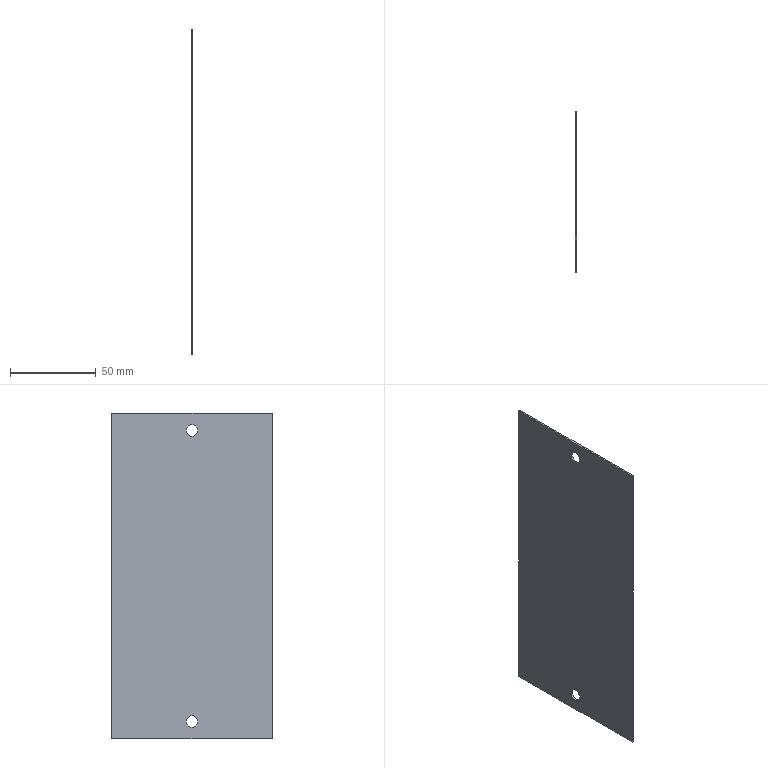Component | SolidWorks | BaseCableHoleBlankingPlate-1 | 1 solid | 10 faces | volume 16005 mm3 | plane 6 | cylinder 4 | commonest cylinder face diameters 7 x4